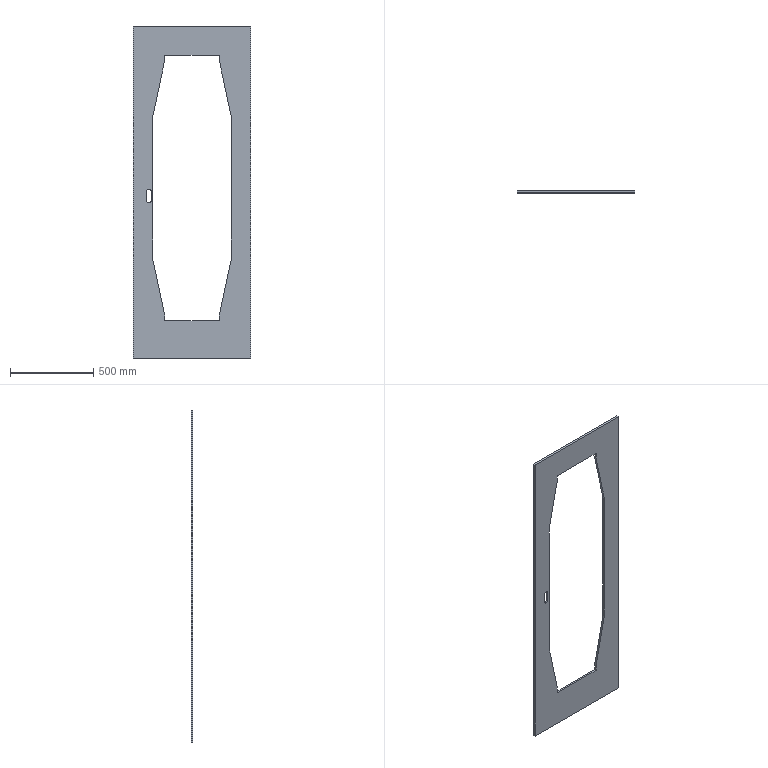Component | NX | CH3404_5-2 | 1 solid | 22 faces | volume 8661518 mm3 | plane 20 | cylinder 2 | commonest cylinder face diameters 30 x2